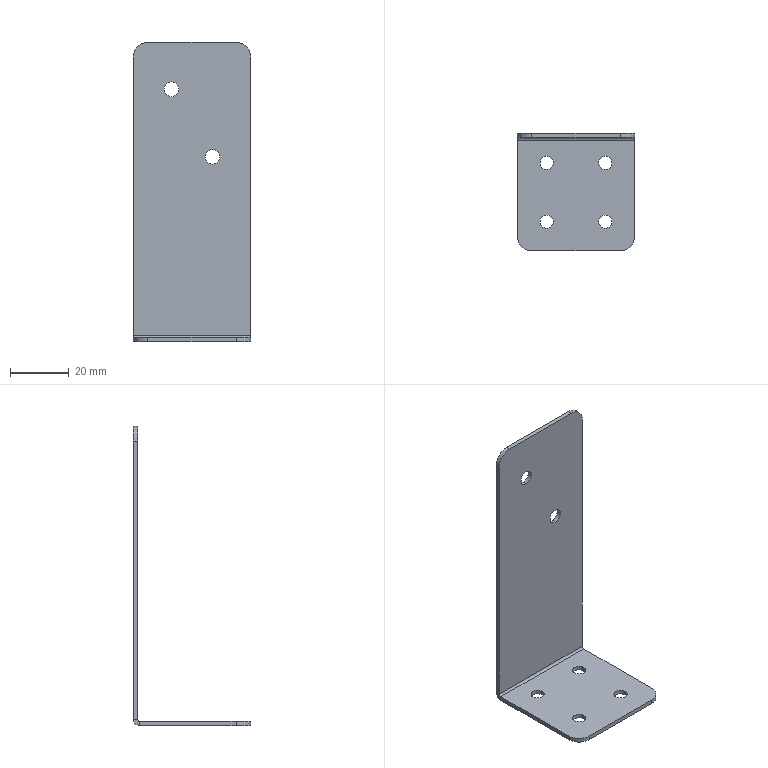Component | SolidWorks | 015-1 | 1 solid | 30 faces | volume 8205 mm3 | cylinder 18 | plane 12 | commonest cylinder face diameters 4.5 x8 5 x4 10 x4 4.473 x1 1.473 x1 | material SUS304